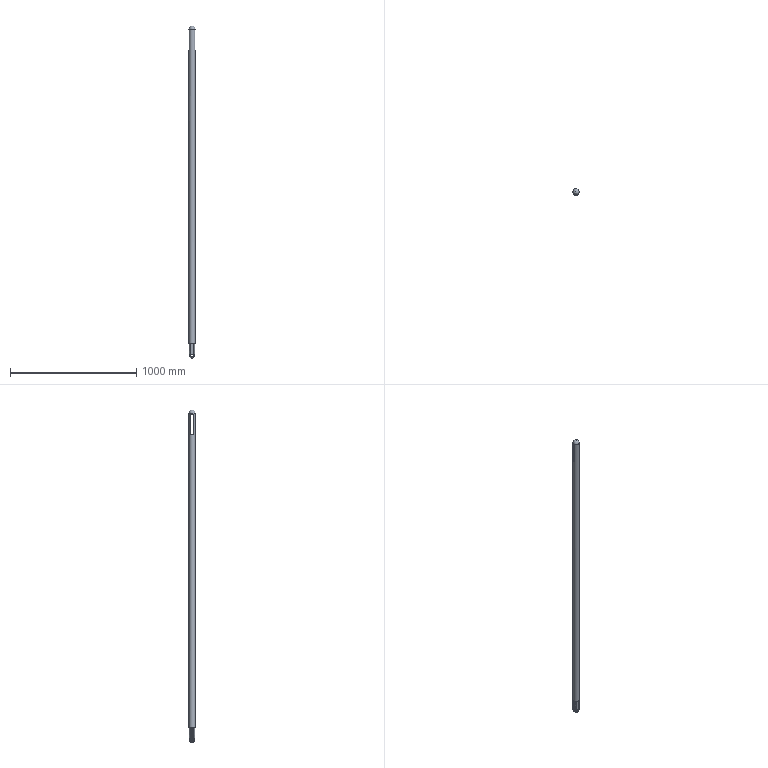Component | NX | MODEL3 | 1 solid | 44 faces | volume 4547304 mm3 | plane 26 | cylinder 11 | spline 6 | sphere 1 | commonest cylinder face diameters 20 x4 40 x2 22 x2 19.955 x2 48.332 x1